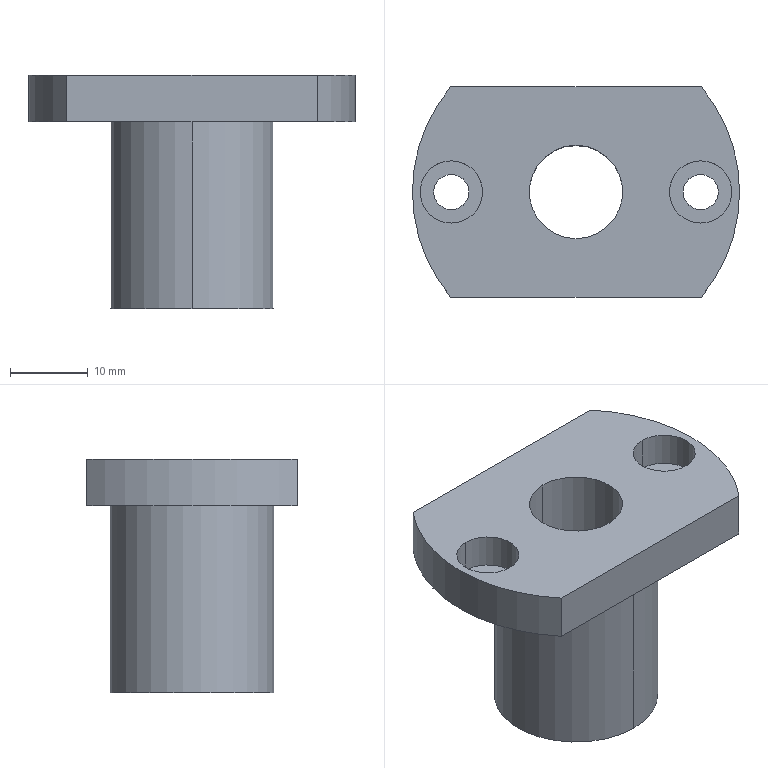Component | SolidWorks | DirectPressureVerticalSeal-1_LMH12UULinearBearing-1 | 1 solid | 21 faces | box 42 x 27 x 30 mm | volume 10727 mm3 | cylinder 14 | plane 7 | commonest cylinder face diameters 8 x4 4.5 x4 12 x2 21 x2 42 x2
build123d program:
from build123d import *

# Parameters (mm, degrees)
BOSS_EXTRUDE1_DEPTH                                 = 6
SKETCH2_W                                           = 24
SKETCH2_H                                           = 10.5
F_12_0_12_DIAMETER_HOLE1_D                          = 12
CYLINDRICAL_COUNTERSUNK_HOLE_FOR_M4_HEX_D           = 4.5
CYLINDRICAL_COUNTERSUNK_HOLE_FOR_M4_HEX_DEPTH       = 30
CYLINDRICAL_COUNTERSUNK_HOLE_FOR_M4_HEX_CBORE_D     = 8
CYLINDRICAL_COUNTERSUNK_HOLE_FOR_M4_HEX_CBORE_DEPTH = 4.4


with BuildPart() as part:
    # Sketch1 → Boss-Extrude1 (new body)
    with BuildSketch(Plane(origin=(6, 0, 0), x_dir=(0, 0, -1), z_dir=(1, 0, 0))):
        with BuildLine():
            Line((13.5, -16.086), (13.5, 16.086))
            ThreePointArc((13.5, 16.086), (0, 21), (-13.5, 16.086))
            Line((-13.5, 16.086), (-13.5, -16.086))
            ThreePointArc((-13.5, -16.086), (0, -21), (13.5, -16.086))
        make_face()
    extrude(amount=-BOSS_EXTRUDE1_DEPTH)

    # Sketch2 → Revolve1 (revolve)
    with BuildSketch(Plane(origin=(0, 0, 0), x_dir=(-1, 0, 0), z_dir=(0, 0, -1)), mode=Mode.PRIVATE) as revolve1_sk:
        with Locations((-18, 5.25)):
            Rectangle(SKETCH2_W, SKETCH2_H)
    revolve(revolve1_sk.sketch.rotate(Axis((30, 0, 0), (-1, 0, 0)), 270), axis=Axis((30, 0, 0), (-1, 0, 0)))

    # 12.0 _12_ Diameter Hole1 (through all)
    with Locations(Plane.ZY):
        with Locations((0, 0)):
            Hole(F_12_0_12_DIAMETER_HOLE1_D / 2)

    # Cylindrical Countersunk Hole for M4 Hex
    with Locations(Plane.ZY):
        with Locations((0, 16), (0, -16)):
            CounterBoreHole(CYLINDRICAL_COUNTERSUNK_HOLE_FOR_M4_HEX_D / 2, CYLINDRICAL_COUNTERSUNK_HOLE_FOR_M4_HEX_CBORE_D / 2, CYLINDRICAL_COUNTERSUNK_HOLE_FOR_M4_HEX_CBORE_DEPTH, depth=CYLINDRICAL_COUNTERSUNK_HOLE_FOR_M4_HEX_DEPTH)


solid = part.part

# Placed as in the assembly
solid = solid.moved(Location((-298.746, 181.873, 324.5), (90, 0, -90)))
STEP:
#1=CARTESIAN_POINT('',(-11.132,7.318,12.602));
#2=VERTEX_POINT('',#1);
#3=CARTESIAN_POINT('',(-11.132,7.003,12.602));
#4=VERTEX_POINT('',#3);
#5=CARTESIAN_POINT('',(-11.132,7.16,12.602));
#6=DIRECTION('',(-0.,-0.,1.));
#7=DIRECTION('',(0.,-1.,0.));
#8=AXIS2_PLACEMENT_3D('',#5,#6,#7);
#9=CIRCLE('',#8,0.1575);
#10=EDGE_CURVE('',#2,#4,#9,.T.);
#11=ORIENTED_EDGE('',*,*,#10,.F.);
#12=CARTESIAN_POINT('',(-11.132,7.318,12.776));
#13=VERTEX_POINT('',#12);
#14=CARTESIAN_POINT('',(-11.132,7.318,12.776));
#15=DIRECTION('',(-0.,-0.,1.));
#16=VECTOR('',#15,39.37);
#17=LINE('',#14,#16);
#18=EDGE_CURVE('',#2,#13,#17,.T.);
#19=ORIENTED_EDGE('',*,*,#18,.T.);
#20=CARTESIAN_POINT('',(-11.132,7.003,12.776));
#21=VERTEX_POINT('',#20);
#22=CARTESIAN_POINT('',(-11.132,7.16,12.776));
#23=DIRECTION('',(-0.,-0.,1.));
#24=DIRECTION('',(0.,-1.,0.));
#25=AXIS2_PLACEMENT_3D('',#22,#23,#24);
#26=CIRCLE('',#25,0.1575);
#27=EDGE_CURVE('',#13,#21,#26,.T.);
#28=ORIENTED_EDGE('',*,*,#27,.T.);
#29=CARTESIAN_POINT('',(-11.132,7.003,12.776));
#30=DIRECTION('',(-0.,-0.,1.));
#31=VECTOR('',#30,39.37);
#32=LINE('',#29,#31);
#33=EDGE_CURVE('',#4,#21,#32,.T.);
#34=ORIENTED_EDGE('',*,*,#33,.F.);
#35=EDGE_LOOP('',(#11,#19,#28,#34));
#36=FACE_OUTER_BOUND('',#35,.T.);
#37=CARTESIAN_POINT('',(-11.132,7.16,12.776));
#38=DIRECTION('',(-0.,-0.,1.));
#39=DIRECTION('',(0.,-1.,0.));
#40=AXIS2_PLACEMENT_3D('',#37,#38,#39);
#41=CYLINDRICAL_SURFACE('',#40,0.1575);
#42=ADVANCED_FACE('',(#36),#41,.F.);
#43=CARTESIAN_POINT('',(-11.132,7.072,12.539));
#44=VERTEX_POINT('',#43);
#45=CARTESIAN_POINT('',(-11.132,7.249,12.539));
#46=VERTEX_POINT('',#45);
#47=CARTESIAN_POINT('',(-11.132,7.16,12.539));
#48=DIRECTION('',(0.,0.,-1.));
#49=DIRECTION('',(0.,1.,0.));
#50=AXIS2_PLACEMENT_3D('',#47,#48,#49);
#51=CIRCLE('',#50,0.08858);
#52=EDGE_CURVE('',#44,#46,#51,.T.);
#53=ORIENTED_EDGE('',*,*,#52,.T.);
#54=CARTESIAN_POINT('',(-11.132,7.249,12.602));
#55=VERTEX_POINT('',#54);
#56=CARTESIAN_POINT('',(-11.132,7.249,12.776));
#57=DIRECTION('',(-0.,-0.,1.));
#58=VECTOR('',#57,39.37);
#59=LINE('',#56,#58);
#60=EDGE_CURVE('',#46,#55,#59,.T.);
#61=ORIENTED_EDGE('',*,*,#60,.T.);
#62=CARTESIAN_POINT('',(-11.132,7.072,12.602));
#63=VERTEX_POINT('',#62);
#64=CARTESIAN_POINT('',(-11.132,7.16,12.602));
#65=DIRECTION('',(-0.,-0.,1.));
#66=DIRECTION('',(0.,-1.,0.));
#67=AXIS2_PLACEMENT_3D('',#64,#65,#66);
#68=CIRCLE('',#67,0.08858);
#69=EDGE_CURVE('',#55,#63,#68,.T.);
#70=ORIENTED_EDGE('',*,*,#69,.T.);
#71=CARTESIAN_POINT('',(-11.132,7.072,12.776));
#72=DIRECTION('',(-0.,-0.,1.));
#73=VECTOR('',#72,39.37);
#74=LINE('',#71,#73);
#75=EDGE_CURVE('',#44,#63,#74,.T.);
#76=ORIENTED_EDGE('',*,*,#75,.F.);
#77=EDGE_LOOP('',(#53,#61,#70,#76));
#78=FACE_OUTER_BOUND('',#77,.T.);
#79=CARTESIAN_POINT('',(-11.132,7.16,12.776));
#80=DIRECTION('',(-0.,-0.,1.));
#81=DIRECTION('',(0.,-1.,0.));
#82=AXIS2_PLACEMENT_3D('',#79,#80,#81);
#83=CYLINDRICAL_SURFACE('',#82,0.08858);
#84=ADVANCED_FACE('',(#78),#83,.F.);
#85=CARTESIAN_POINT('',(-12.392,7.318,12.602));
#86=VERTEX_POINT('',#85);
#87=CARTESIAN_POINT('',(-12.392,7.003,12.602));
#88=VERTEX_POINT('',#87);
#89=CARTESIAN_POINT('',(-12.392,7.16,12.602));
#90=DIRECTION('',(-0.,-0.,1.));
#91=DIRECTION('',(0.,-1.,0.));
#92=AXIS2_PLACEMENT_3D('',#89,#90,#91);
#93=CIRCLE('',#92,0.1575);
#94=EDGE_CURVE('',#86,#88,#93,.T.);
#95=ORIENTED_EDGE('',*,*,#94,.F.);
#96=CARTESIAN_POINT('',(-12.392,7.318,12.776));
#97=VERTEX_POINT('',#96);
#98=CARTESIAN_POINT('',(-12.392,7.318,12.776));
#99=DIRECTION('',(-0.,-0.,1.));
#100=VECTOR('',#99,39.37);
#101=LINE('',#98,#100);
#102=EDGE_CURVE('',#86,#97,#101,.T.);
#103=ORIENTED_EDGE('',*,*,#102,.T.);
#104=CARTESIAN_POINT('',(-12.392,7.003,12.776));
#105=VERTEX_POINT('',#104);
#106=CARTESIAN_POINT('',(-12.392,7.16,12.776));
#107=DIRECTION('',(-0.,-0.,1.));
#108=DIRECTION('',(0.,-1.,0.));
#109=AXIS2_PLACEMENT_3D('',#106,#107,#108);
#110=CIRCLE('',#109,0.1575);
#111=EDGE_CURVE('',#97,#105,#110,.T.);
#112=ORIENTED_EDGE('',*,*,#111,.T.);
#113=CARTESIAN_POINT('',(-12.392,7.003,12.776));
#114=DIRECTION('',(-0.,-0.,1.));
#115=VECTOR('',#114,39.37);
#116=LINE('',#113,#115);
#117=EDGE_CURVE('',#88,#105,#116,.T.);
#118=ORIENTED_EDGE('',*,*,#117,.F.);
#119=EDGE_LOOP('',(#95,#103,#112,#118));
#120=FACE_OUTER_BOUND('',#119,.T.);
#121=CARTESIAN_POINT('',(-12.392,7.16,12.776));
#122=DIRECTION('',(-0.,-0.,1.));
#123=DIRECTION('',(0.,-1.,0.));
#124=AXIS2_PLACEMENT_3D('',#121,#122,#123);
#125=CYLINDRICAL_SURFACE('',#124,0.1575);
#126=ADVANCED_FACE('',(#120),#125,.F.);
#127=CARTESIAN_POINT('',(-12.392,7.072,12.539));
#128=VERTEX_POINT('',#127);
#129=CARTESIAN_POINT('',(-12.392,7.249,12.539));
#130=VERTEX_POINT('',#129);
#131=CARTESIAN_POINT('',(-12.392,7.16,12.539));
#132=DIRECTION('',(0.,0.,-1.));
#133=DIRECTION('',(0.,1.,0.));
#134=AXIS2_PLACEMENT_3D('',#131,#132,#133);
#135=CIRCLE('',#134,0.08858);
#136=EDGE_CURVE('',#128,#130,#135,.T.);
#137=ORIENTED_EDGE('',*,*,#136,.T.);
#138=CARTESIAN_POINT('',(-12.392,7.249,12.602));
#139=VERTEX_POINT('',#138);
#140=CARTESIAN_POINT('',(-12.392,7.249,12.776));
#141=DIRECTION('',(-0.,-0.,1.));
#142=VECTOR('',#141,39.37);
#143=LINE('',#140,#142);
#144=EDGE_CURVE('',#130,#139,#143,.T.);
#145=ORIENTED_EDGE('',*,*,#144,.T.);
#146=CARTESIAN_POINT('',(-12.392,7.072,12.602));
#147=VERTEX_POINT('',#146);
#148=CARTESIAN_POINT('',(-12.392,7.16,12.602));
#149=DIRECTION('',(-0.,-0.,1.));
#150=DIRECTION('',(0.,-1.,0.));
#151=AXIS2_PLACEMENT_3D('',#148,#149,#150);
#152=CIRCLE('',#151,0.08858);
#153=EDGE_CURVE('',#139,#147,#152,.T.);
#154=ORIENTED_EDGE('',*,*,#153,.T.);
#155=CARTESIAN_POINT('',(-12.392,7.072,12.776));
#156=DIRECTION('',(-0.,-0.,1.));
#157=VECTOR('',#156,39.37);
#158=LINE('',#155,#157);
#159=EDGE_CURVE('',#128,#147,#158,.T.);
#160=ORIENTED_EDGE('',*,*,#159,.F.);
#161=EDGE_LOOP('',(#137,#145,#154,#160));
#162=FACE_OUTER_BOUND('',#161,.T.);
#163=CARTESIAN_POINT('',(-12.392,7.16,12.776));
#164=DIRECTION('',(-0.,-0.,1.));
#165=DIRECTION('',(0.,-1.,0.));
#166=AXIS2_PLACEMENT_3D('',#163,#164,#165);
#167=CYLINDRICAL_SURFACE('',#166,0.08858);
#168=ADVANCED_FACE('',(#162),#167,.F.);
#169=CARTESIAN_POINT('',(-11.762,7.397,11.594));
#170=VERTEX_POINT('',#169);
#171=CARTESIAN_POINT('',(-11.762,6.924,11.594));
#172=VERTEX_POINT('',#171);
#173=CARTESIAN_POINT('',(-11.762,7.16,11.594));
#174=DIRECTION('',(-0.,-0.,1.));
#175=DIRECTION('',(0.,-1.,0.));
#176=AXIS2_PLACEMENT_3D('',#173,#174,#175);
#177=CIRCLE('',#176,0.2362);
#178=EDGE_CURVE('',#170,#172,#177,.T.);
#179=ORIENTED_EDGE('',*,*,#178,.F.);
#180=CARTESIAN_POINT('',(-11.762,7.397,12.776));
#181=VERTEX_POINT('',#180);
#182=CARTESIAN_POINT('',(-11.762,7.397,12.776));
#183=DIRECTION('',(-0.,-0.,1.));
#184=VECTOR('',#183,39.37);
#185=LINE('',#182,#184);
#186=EDGE_CURVE('',#170,#181,#185,.T.);
#187=ORIENTED_EDGE('',*,*,#186,.T.);
#188=CARTESIAN_POINT('',(-11.762,6.924,12.776));
#189=VERTEX_POINT('',#188);
#190=CARTESIAN_POINT('',(-11.762,7.16,12.776));
#191=DIRECTION('',(-0.,-0.,1.));
#192=DIRECTION('',(0.,-1.,0.));
#193=AXIS2_PLACEMENT_3D('',#190,#191,#192);
#194=CIRCLE('',#193,0.2362);
#195=EDGE_CURVE('',#181,#189,#194,.T.);
#196=ORIENTED_EDGE('',*,*,#195,.T.);
#197=CARTESIAN_POINT('',(-11.762,6.924,12.776));
#198=DIRECTION('',(-0.,-0.,1.));
#199=VECTOR('',#198,39.37);
#200=LINE('',#197,#199);
#201=EDGE_CURVE('',#172,#189,#200,.T.);
#202=ORIENTED_EDGE('',*,*,#201,.F.);
#203=EDGE_LOOP('',(#179,#187,#196,#202));
#204=FACE_OUTER_BOUND('',#203,.T.);
#205=CARTESIAN_POINT('',(-11.762,7.16,12.776));
#206=DIRECTION('',(-0.,-0.,1.));
#207=DIRECTION('',(0.,-1.,0.));
#208=AXIS2_PLACEMENT_3D('',#205,#206,#207);
#209=CYLINDRICAL_SURFACE('',#208,0.2362);
#210=ADVANCED_FACE('',(#204),#209,.F.);
#211=CARTESIAN_POINT('',(-11.762,6.747,11.594));
#212=VERTEX_POINT('',#211);
#213=CARTESIAN_POINT('',(-11.762,7.574,11.594));
#214=VERTEX_POINT('',#213);
#215=CARTESIAN_POINT('',(-11.762,7.16,11.594));
#216=DIRECTION('',(-0.,-0.,1.));
#217=DIRECTION('',(0.,-1.,0.));
#218=AXIS2_PLACEMENT_3D('',#215,#216,#217);
#219=CIRCLE('',#218,0.4134);
#220=EDGE_CURVE('',#212,#214,#219,.T.);
#221=ORIENTED_EDGE('',*,*,#220,.T.);
#222=CARTESIAN_POINT('',(-11.762,7.574,12.539));
#223=VERTEX_POINT('',#222);
#224=CARTESIAN_POINT('',(-11.762,7.574,11.594));
#225=DIRECTION('',(-0.,-0.,1.));
#226=VECTOR('',#225,39.37);
#227=LINE('',#224,#226);
#228=EDGE_CURVE('',#214,#223,#227,.T.);
#229=ORIENTED_EDGE('',*,*,#228,.T.);
#230=CARTESIAN_POINT('',(-11.762,6.747,12.539));
#231=VERTEX_POINT('',#230);
#232=CARTESIAN_POINT('',(-11.762,7.16,12.539));
#233=DIRECTION('',(-0.,-0.,1.));
#234=DIRECTION('',(0.,-1.,0.));
#235=AXIS2_PLACEMENT_3D('',#232,#233,#234);
#236=CIRCLE('',#235,0.4134);
#237=EDGE_CURVE('',#231,#223,#236,.T.);
#238=ORIENTED_EDGE('',*,*,#237,.F.);
#239=CARTESIAN_POINT('',(-11.762,6.747,11.594));
#240=DIRECTION('',(-0.,-0.,1.));
#241=VECTOR('',#240,39.37);
#242=LINE('',#239,#241);
#243=EDGE_CURVE('',#212,#231,#242,.T.);
#244=ORIENTED_EDGE('',*,*,#243,.F.);
#245=EDGE_LOOP('',(#221,#229,#238,#244));
#246=FACE_OUTER_BOUND('',#245,.T.);
#247=CARTESIAN_POINT('',(-11.762,7.16,11.594));
#248=DIRECTION('',(-0.,-0.,1.));
#249=DIRECTION('',(0.,-1.,0.));
#250=AXIS2_PLACEMENT_3D('',#247,#248,#249);
#251=CYLINDRICAL_SURFACE('',#250,0.4134);
#252=ADVANCED_FACE('',(#246),#251,.T.);
#253=CARTESIAN_POINT('',(-12.395,6.629,12.539));
#254=VERTEX_POINT('',#253);
#255=CARTESIAN_POINT('',(-12.395,7.692,12.539));
#256=VERTEX_POINT('',#255);
#257=CARTESIAN_POINT('',(-11.762,7.16,12.539));
#258=DIRECTION('',(0.,0.,-1.));
#259=DIRECTION('',(0.,1.,0.));
#260=AXIS2_PLACEMENT_3D('',#257,#258,#259);
#261=CIRCLE('',#260,0.8268);
#262=EDGE_CURVE('',#254,#256,#261,.T.);
#263=ORIENTED_EDGE('',*,*,#262,.F.);
#264=CARTESIAN_POINT('',(-12.395,6.629,12.776));
#265=VERTEX_POINT('',#264);
#266=CARTESIAN_POINT('',(-12.395,6.629,12.776));
#267=DIRECTION('',(0.,0.,-1.));
#268=VECTOR('',#267,39.37);
#269=LINE('',#266,#268);
#270=EDGE_CURVE('',#265,#254,#269,.T.);
#271=ORIENTED_EDGE('',*,*,#270,.F.);
#272=CARTESIAN_POINT('',(-12.395,7.692,12.776));
#273=VERTEX_POINT('',#272);
#274=CARTESIAN_POINT('',(-11.762,7.16,12.776));
#275=DIRECTION('',(0.,0.,-1.));
#276=DIRECTION('',(0.,1.,0.));
#277=AXIS2_PLACEMENT_3D('',#274,#275,#276);
#278=CIRCLE('',#277,0.8268);
#279=EDGE_CURVE('',#265,#273,#278,.T.);
#280=ORIENTED_EDGE('',*,*,#279,.T.);
#281=CARTESIAN_POINT('',(-12.395,7.692,12.776));
#282=DIRECTION('',(0.,0.,-1.));
#283=VECTOR('',#282,39.37);
#284=LINE('',#281,#283);
#285=EDGE_CURVE('',#273,#256,#284,.T.);
#286=ORIENTED_EDGE('',*,*,#285,.T.);
#287=EDGE_LOOP('',(#263,#271,#280,#286));
#288=FACE_OUTER_BOUND('',#287,.T.);
#289=CARTESIAN_POINT('',(-11.762,7.16,12.776));
#290=DIRECTION('',(0.,0.,-1.));
#291=DIRECTION('',(0.,1.,0.));
#292=AXIS2_PLACEMENT_3D('',#289,#290,#291);
#293=CYLINDRICAL_SURFACE('',#292,0.8268);
#294=ADVANCED_FACE('',(#288),#293,.T.);
#295=CARTESIAN_POINT('',(-11.128,6.629,12.539));
#296=VERTEX_POINT('',#295);
#297=CARTESIAN_POINT('',(-11.128,6.629,12.539));
#298=DIRECTION('',(-1.,-0.,-0.));
#299=VECTOR('',#298,39.37);
#300=LINE('',#297,#299);
#301=EDGE_CURVE('',#296,#254,#300,.T.);
#302=ORIENTED_EDGE('',*,*,#301,.F.);
#303=CARTESIAN_POINT('',(-11.128,6.629,12.776));
#304=VERTEX_POINT('',#303);
#305=CARTESIAN_POINT('',(-11.128,6.629,12.776));
#306=DIRECTION('',(0.,0.,-1.));
#307=VECTOR('',#306,39.37);
#308=LINE('',#305,#307);
#309=EDGE_CURVE('',#304,#296,#308,.T.);
#310=ORIENTED_EDGE('',*,*,#309,.F.);
#311=CARTESIAN_POINT('',(-11.128,6.629,12.776));
#312=DIRECTION('',(-1.,-0.,-0.));
#313=VECTOR('',#312,39.37);
#314=LINE('',#311,#313);
#315=EDGE_CURVE('',#304,#265,#314,.T.);
#316=ORIENTED_EDGE('',*,*,#315,.T.);
#317=ORIENTED_EDGE('',*,*,#270,.T.);
#318=EDGE_LOOP('',(#302,#310,#316,#317));
#319=FACE_OUTER_BOUND('',#318,.T.);
#320=CARTESIAN_POINT('',(-11.128,6.629,12.776));
#321=DIRECTION('',(0.,-1.,-0.));
#322=DIRECTION('',(0.,0.,-1.));
#323=AXIS2_PLACEMENT_3D('',#320,#321,#322);
#324=PLANE('',#323);
#325=ADVANCED_FACE('',(#319),#324,.T.);
#326=CARTESIAN_POINT('',(-11.128,7.692,12.539));
#327=VERTEX_POINT('',#326);
#328=CARTESIAN_POINT('',(-11.762,7.16,12.539));
#329=DIRECTION('',(0.,0.,-1.));
#330=DIRECTION('',(0.,1.,0.));
#331=AXIS2_PLACEMENT_3D('',#328,#329,#330);
#332=CIRCLE('',#331,0.8268);
#333=EDGE_CURVE('',#327,#296,#332,.T.);
#334=ORIENTED_EDGE('',*,*,#333,.F.);
#335=CARTESIAN_POINT('',(-11.128,7.692,12.776));
#336=VERTEX_POINT('',#335);
#337=CARTESIAN_POINT('',(-11.128,7.692,12.776));
#338=DIRECTION('',(0.,0.,-1.));
#339=VECTOR('',#338,39.37);
#340=LINE('',#337,#339);
#341=EDGE_CURVE('',#336,#327,#340,.T.);
#342=ORIENTED_EDGE('',*,*,#341,.F.);
#343=CARTESIAN_POINT('',(-11.762,7.16,12.776));
#344=DIRECTION('',(0.,0.,-1.));
#345=DIRECTION('',(0.,1.,0.));
#346=AXIS2_PLACEMENT_3D('',#343,#344,#345);
#347=CIRCLE('',#346,0.8268);
#348=EDGE_CURVE('',#336,#304,#347,.T.);
#349=ORIENTED_EDGE('',*,*,#348,.T.);
#350=ORIENTED_EDGE('',*,*,#309,.T.);
#351=EDGE_LOOP('',(#334,#342,#349,#350));
#352=FACE_OUTER_BOUND('',#351,.T.);
#353=CARTESIAN_POINT('',(-11.762,7.16,12.776));
#354=DIRECTION('',(0.,0.,-1.));
#355=DIRECTION('',(0.,1.,0.));
#356=AXIS2_PLACEMENT_3D('',#353,#354,#355);
#357=CYLINDRICAL_SURFACE('',#356,0.8268);
#358=ADVANCED_FACE('',(#352),#357,.T.);
#359=CARTESIAN_POINT('',(-12.395,7.692,12.539));
#360=DIRECTION('',(1.,0.,0.));
#361=VECTOR('',#360,39.37);
#362=LINE('',#359,#361);
#363=EDGE_CURVE('',#256,#327,#362,.T.);
#364=ORIENTED_EDGE('',*,*,#363,.F.);
#365=ORIENTED_EDGE('',*,*,#285,.F.);
#366=CARTESIAN_POINT('',(-12.395,7.692,12.776));
#367=DIRECTION('',(1.,0.,0.));
#368=VECTOR('',#367,39.37);
#369=LINE('',#366,#368);
#370=EDGE_CURVE('',#273,#336,#369,.T.);
#371=ORIENTED_EDGE('',*,*,#370,.T.);
#372=ORIENTED_EDGE('',*,*,#341,.T.);
#373=EDGE_LOOP('',(#364,#365,#371,#372));
#374=FACE_OUTER_BOUND('',#373,.T.);
#375=CARTESIAN_POINT('',(-12.395,7.692,12.776));
#376=DIRECTION('',(-0.,1.,0.));
#377=DIRECTION('',(1.,0.,0.));
#378=AXIS2_PLACEMENT_3D('',#375,#376,#377);
#379=PLANE('',#378);
#380=ADVANCED_FACE('',(#374),#379,.T.);
#381=CARTESIAN_POINT('',(-11.132,7.16,12.776));
#382=DIRECTION('',(-0.,-0.,1.));
#383=DIRECTION('',(0.,-1.,0.));
#384=AXIS2_PLACEMENT_3D('',#381,#382,#383);
#385=CIRCLE('',#384,0.1575);
#386=EDGE_CURVE('',#21,#13,#385,.T.);
#387=ORIENTED_EDGE('',*,*,#386,.F.);
#388=ORIENTED_EDGE('',*,*,#27,.F.);
#389=EDGE_LOOP('',(#387,#388));
#390=FACE_BOUND('',#389,.T.);
#391=CARTESIAN_POINT('',(-12.392,7.16,12.776));
#392=DIRECTION('',(-0.,-0.,1.));
#393=DIRECTION('',(0.,-1.,0.));
#394=AXIS2_PLACEMENT_3D('',#391,#392,#393);
#395=CIRCLE('',#394,0.1575);
#396=EDGE_CURVE('',#105,#97,#395,.T.);
#397=ORIENTED_EDGE('',*,*,#396,.F.);
#398=ORIENTED_EDGE('',*,*,#111,.F.);
#399=EDGE_LOOP('',(#397,#398));
#400=FACE_BOUND('',#399,.T.);
#401=CARTESIAN_POINT('',(-11.762,7.16,12.776));
#402=DIRECTION('',(-0.,-0.,1.));
#403=DIRECTION('',(0.,-1.,0.));
#404=AXIS2_PLACEMENT_3D('',#401,#402,#403);
#405=CIRCLE('',#404,0.2362);
#406=EDGE_CURVE('',#189,#181,#405,.T.);
#407=ORIENTED_EDGE('',*,*,#406,.F.);
#408=ORIENTED_EDGE('',*,*,#195,.F.);
#409=EDGE_LOOP('',(#407,#408));
#410=FACE_BOUND('',#409,.T.);
#411=ORIENTED_EDGE('',*,*,#279,.F.);
#412=ORIENTED_EDGE('',*,*,#315,.F.);
#413=ORIENTED_EDGE('',*,*,#348,.F.);
#414=ORIENTED_EDGE('',*,*,#370,.F.);
#415=EDGE_LOOP('',(#411,#412,#413,#414));
#416=FACE_OUTER_BOUND('',#415,.T.);
#417=CARTESIAN_POINT('',(-11.762,7.16,12.776));
#418=DIRECTION('',(0.,0.,-1.));
#419=DIRECTION('',(-0.,1.,0.));
#420=AXIS2_PLACEMENT_3D('',#417,#418,#419);
#421=PLANE('',#420);
#422=ADVANCED_FACE('',(#390,#400,#410,#416),#421,.F.);
#423=ORIENTED_EDGE('',*,*,#52,.F.);
#424=CARTESIAN_POINT('',(-11.132,7.16,12.539));
#425=DIRECTION('',(0.,0.,-1.));
#426=DIRECTION('',(0.,1.,0.));
#427=AXIS2_PLACEMENT_3D('',#424,#425,#426);
#428=CIRCLE('',#427,0.08858);
#429=EDGE_CURVE('',#46,#44,#428,.T.);
#430=ORIENTED_EDGE('',*,*,#429,.F.);
#431=EDGE_LOOP('',(#423,#430));
#432=FACE_BOUND('',#431,.T.);
#433=ORIENTED_EDGE('',*,*,#136,.F.);
#434=CARTESIAN_POINT('',(-12.392,7.16,12.539));
#435=DIRECTION('',(0.,0.,-1.));
#436=DIRECTION('',(0.,1.,0.));
#437=AXIS2_PLACEMENT_3D('',#434,#435,#436);
#438=CIRCLE('',#437,0.08858);
#439=EDGE_CURVE('',#130,#128,#438,.T.);
#440=ORIENTED_EDGE('',*,*,#439,.F.);
#441=EDGE_LOOP('',(#433,#440));
#442=FACE_BOUND('',#441,.T.);
#443=ORIENTED_EDGE('',*,*,#237,.T.);
#444=CARTESIAN_POINT('',(-11.762,7.16,12.539));
#445=DIRECTION('',(-0.,-0.,1.));
#446=DIRECTION('',(0.,-1.,0.));
#447=AXIS2_PLACEMENT_3D('',#444,#445,#446);
#448=CIRCLE('',#447,0.4134);
#449=EDGE_CURVE('',#223,#231,#448,.T.);
#450=ORIENTED_EDGE('',*,*,#449,.T.);
#451=EDGE_LOOP('',(#443,#450));
#452=FACE_BOUND('',#451,.T.);
#453=ORIENTED_EDGE('',*,*,#262,.T.);
#454=ORIENTED_EDGE('',*,*,#363,.T.);
#455=ORIENTED_EDGE('',*,*,#333,.T.);
#456=ORIENTED_EDGE('',*,*,#301,.T.);
#457=EDGE_LOOP('',(#453,#454,#455,#456));
#458=FACE_OUTER_BOUND('',#457,.T.);
#459=CARTESIAN_POINT('',(-11.762,7.16,12.539));
#460=DIRECTION('',(0.,0.,-1.));
#461=DIRECTION('',(-0.,1.,0.));
#462=AXIS2_PLACEMENT_3D('',#459,#460,#461);
#463=PLANE('',#462);
#464=ADVANCED_FACE('',(#432,#442,#452,#458),#463,.T.);
#465=ORIENTED_EDGE('',*,*,#228,.F.);
#466=CARTESIAN_POINT('',(-11.762,7.16,11.594));
#467=DIRECTION('',(-0.,-0.,1.));
#468=DIRECTION('',(0.,-1.,0.));
#469=AXIS2_PLACEMENT_3D('',#466,#467,#468);
#470=CIRCLE('',#469,0.4134);
#471=EDGE_CURVE('',#214,#212,#470,.T.);
#472=ORIENTED_EDGE('',*,*,#471,.T.);
#473=ORIENTED_EDGE('',*,*,#243,.T.);
#474=ORIENTED_EDGE('',*,*,#449,.F.);
#475=EDGE_LOOP('',(#465,#472,#473,#474));
#476=FACE_OUTER_BOUND('',#475,.T.);
#477=CARTESIAN_POINT('',(-11.762,7.16,11.594));
#478=DIRECTION('',(-0.,-0.,1.));
#479=DIRECTION('',(0.,-1.,0.));
#480=AXIS2_PLACEMENT_3D('',#477,#478,#479);
#481=CYLINDRICAL_SURFACE('',#480,0.4134);
#482=ADVANCED_FACE('',(#476),#481,.T.);
#483=CARTESIAN_POINT('',(-11.762,7.16,11.594));
#484=DIRECTION('',(-0.,-0.,1.));
#485=DIRECTION('',(0.,-1.,0.));
#486=AXIS2_PLACEMENT_3D('',#483,#484,#485);
#487=CIRCLE('',#486,0.2362);
#488=EDGE_CURVE('',#172,#170,#487,.T.);
#489=ORIENTED_EDGE('',*,*,#488,.T.);
#490=ORIENTED_EDGE('',*,*,#178,.T.);
#491=EDGE_LOOP('',(#489,#490));
#492=FACE_BOUND('',#491,.T.);
#493=ORIENTED_EDGE('',*,*,#220,.F.);
#494=ORIENTED_EDGE('',*,*,#471,.F.);
#495=EDGE_LOOP('',(#493,#494));
#496=FACE_OUTER_BOUND('',#495,.T.);
#497=CARTESIAN_POINT('',(-11.348,7.16,11.594));
#498=DIRECTION('',(0.,0.,-1.));
#499=DIRECTION('',(-0.,1.,0.));
#500=AXIS2_PLACEMENT_3D('',#497,#498,#499);
#501=PLANE('',#500);
#502=ADVANCED_FACE('',(#492,#496),#501,.T.);
#503=ORIENTED_EDGE('',*,*,#186,.F.);
#504=ORIENTED_EDGE('',*,*,#488,.F.);
#505=ORIENTED_EDGE('',*,*,#201,.T.);
#506=ORIENTED_EDGE('',*,*,#406,.T.);
#507=EDGE_LOOP('',(#503,#504,#505,#506));
#508=FACE_OUTER_BOUND('',#507,.T.);
#509=CARTESIAN_POINT('',(-11.762,7.16,12.776));
#510=DIRECTION('',(-0.,-0.,1.));
#511=DIRECTION('',(0.,-1.,0.));
#512=AXIS2_PLACEMENT_3D('',#509,#510,#511);
#513=CYLINDRICAL_SURFACE('',#512,0.2362);
#514=ADVANCED_FACE('',(#508),#513,.F.);
#515=ORIENTED_EDGE('',*,*,#144,.F.);
#516=ORIENTED_EDGE('',*,*,#439,.T.);
#517=ORIENTED_EDGE('',*,*,#159,.T.);
#518=CARTESIAN_POINT('',(-12.392,7.16,12.602));
#519=DIRECTION('',(-0.,-0.,1.));
#520=DIRECTION('',(0.,-1.,0.));
#521=AXIS2_PLACEMENT_3D('',#518,#519,#520);
#522=CIRCLE('',#521,0.08858);
#523=EDGE_CURVE('',#147,#139,#522,.T.);
#524=ORIENTED_EDGE('',*,*,#523,.T.);
#525=EDGE_LOOP('',(#515,#516,#517,#524));
#526=FACE_OUTER_BOUND('',#525,.T.);
#527=CARTESIAN_POINT('',(-12.392,7.16,12.776));
#528=DIRECTION('',(-0.,-0.,1.));
#529=DIRECTION('',(0.,-1.,0.));
#530=AXIS2_PLACEMENT_3D('',#527,#528,#529);
#531=CYLINDRICAL_SURFACE('',#530,0.08858);
#532=ADVANCED_FACE('',(#526),#531,.F.);
#533=ORIENTED_EDGE('',*,*,#523,.F.);
#534=ORIENTED_EDGE('',*,*,#153,.F.);
#535=EDGE_LOOP('',(#533,#534));
#536=FACE_BOUND('',#535,.T.);
#537=CARTESIAN_POINT('',(-12.392,7.16,12.602));
#538=DIRECTION('',(-0.,-0.,1.));
#539=DIRECTION('',(0.,-1.,0.));
#540=AXIS2_PLACEMENT_3D('',#537,#538,#539);
#541=CIRCLE('',#540,0.1575);
#542=EDGE_CURVE('',#88,#86,#541,.T.);
#543=ORIENTED_EDGE('',*,*,#542,.T.);
#544=ORIENTED_EDGE('',*,*,#94,.T.);
#545=EDGE_LOOP('',(#543,#544));
#546=FACE_OUTER_BOUND('',#545,.T.);
#547=CARTESIAN_POINT('',(-12.303,7.16,12.602));
#548=DIRECTION('',(0.,0.,-1.));
#549=DIRECTION('',(-0.,1.,0.));
#550=AXIS2_PLACEMENT_3D('',#547,#548,#549);
#551=PLANE('',#550);
#552=ADVANCED_FACE('',(#536,#546),#551,.F.);
#553=ORIENTED_EDGE('',*,*,#102,.F.);
#554=ORIENTED_EDGE('',*,*,#542,.F.);
#555=ORIENTED_EDGE('',*,*,#117,.T.);
#556=ORIENTED_EDGE('',*,*,#396,.T.);
#557=EDGE_LOOP('',(#553,#554,#555,#556));
#558=FACE_OUTER_BOUND('',#557,.T.);
#559=CARTESIAN_POINT('',(-12.392,7.16,12.776));
#560=DIRECTION('',(-0.,-0.,1.));
#561=DIRECTION('',(0.,-1.,0.));
#562=AXIS2_PLACEMENT_3D('',#559,#560,#561);
#563=CYLINDRICAL_SURFACE('',#562,0.1575);
#564=ADVANCED_FACE('',(#558),#563,.F.);
#565=ORIENTED_EDGE('',*,*,#60,.F.);
#566=ORIENTED_EDGE('',*,*,#429,.T.);
#567=ORIENTED_EDGE('',*,*,#75,.T.);
#568=CARTESIAN_POINT('',(-11.132,7.16,12.602));
#569=DIRECTION('',(-0.,-0.,1.));
#570=DIRECTION('',(0.,-1.,0.));
#571=AXIS2_PLACEMENT_3D('',#568,#569,#570);
#572=CIRCLE('',#571,0.08858);
#573=EDGE_CURVE('',#63,#55,#572,.T.);
#574=ORIENTED_EDGE('',*,*,#573,.T.);
#575=EDGE_LOOP('',(#565,#566,#567,#574));
#576=FACE_OUTER_BOUND('',#575,.T.);
#577=CARTESIAN_POINT('',(-11.132,7.16,12.776));
#578=DIRECTION('',(-0.,-0.,1.));
#579=DIRECTION('',(0.,-1.,0.));
#580=AXIS2_PLACEMENT_3D('',#577,#578,#579);
#581=CYLINDRICAL_SURFACE('',#580,0.08858);
#582=ADVANCED_FACE('',(#576),#581,.F.);
#583=ORIENTED_EDGE('',*,*,#573,.F.);
#584=ORIENTED_EDGE('',*,*,#69,.F.);
#585=EDGE_LOOP('',(#583,#584));
#586=FACE_BOUND('',#585,.T.);
#587=CARTESIAN_POINT('',(-11.132,7.16,12.602));
#588=DIRECTION('',(-0.,-0.,1.));
#589=DIRECTION('',(0.,-1.,0.));
#590=AXIS2_PLACEMENT_3D('',#587,#588,#589);
#591=CIRCLE('',#590,0.1575);
#592=EDGE_CURVE('',#4,#2,#591,.T.);
#593=ORIENTED_EDGE('',*,*,#592,.T.);
#594=ORIENTED_EDGE('',*,*,#10,.T.);
#595=EDGE_LOOP('',(#593,#594));
#596=FACE_OUTER_BOUND('',#595,.T.);
#597=CARTESIAN_POINT('',(-11.043,7.16,12.602));
#598=DIRECTION('',(0.,0.,-1.));
#599=DIRECTION('',(-0.,1.,0.));
#600=AXIS2_PLACEMENT_3D('',#597,#598,#599);
#601=PLANE('',#600);
#602=ADVANCED_FACE('',(#586,#596),#601,.F.);
#603=ORIENTED_EDGE('',*,*,#18,.F.);
#604=ORIENTED_EDGE('',*,*,#592,.F.);
#605=ORIENTED_EDGE('',*,*,#33,.T.);
#606=ORIENTED_EDGE('',*,*,#386,.T.);
#607=EDGE_LOOP('',(#603,#604,#605,#606));
#608=FACE_OUTER_BOUND('',#607,.T.);
#609=CARTESIAN_POINT('',(-11.132,7.16,12.776));
#610=DIRECTION('',(-0.,-0.,1.));
#611=DIRECTION('',(0.,-1.,0.));
#612=AXIS2_PLACEMENT_3D('',#609,#610,#611);
#613=CYLINDRICAL_SURFACE('',#612,0.1575);
#614=ADVANCED_FACE('',(#608),#613,.F.);
#615=CLOSED_SHELL('',(#42,#84,#126,#168,#210,#252,#294,#325,#358,#380,#422,#464,#482,#502,#514,#532,#552,#564,#582,#602,#614));
#616=MANIFOLD_SOLID_BREP('',#615);
#617=CARTESIAN_POINT('',(0.,0.,0.));
#618=DIRECTION('',(0.,0.,1.));
#619=DIRECTION('',(1.,0.,0.));
#620=AXIS2_PLACEMENT_3D('',#617,#618,#619);
#621=(LENGTH_UNIT()NAMED_UNIT(*)SI_UNIT($,.METRE.));
#622=LENGTH_MEASURE_WITH_UNIT(LENGTH_MEASURE(0.0254),#621);
#623=DIMENSIONAL_EXPONENTS(1.,0.,0.,0.,0.,0.,0.);
#624=(CONVERSION_BASED_UNIT('',#622)LENGTH_UNIT()NAMED_UNIT(#623));
#625=UNCERTAINTY_MEASURE_WITH_UNIT(LENGTH_MEASURE(0.00001),#624,'','');
#626=(NAMED_UNIT(*)PLANE_ANGLE_UNIT()SI_UNIT($,.RADIAN.));
#627=(NAMED_UNIT(*)SI_UNIT($,.STERADIAN.)SOLID_ANGLE_UNIT());
#628=(GEOMETRIC_REPRESENTATION_CONTEXT(3)GLOBAL_UNCERTAINTY_ASSIGNED_CONTEXT((#625))GLOBAL_UNIT_ASSIGNED_CONTEXT((#624,#626,#627))REPRESENTATION_CONTEXT('',''));
#629=ADVANCED_BREP_SHAPE_REPRESENTATION('',(#616,#620),#628);
#630=COLOUR_RGB('',0.7922,0.8196,0.9333);
#631=FILL_AREA_STYLE_COLOUR('',#630);
#632=FILL_AREA_STYLE('',(#631));
#633=SURFACE_STYLE_FILL_AREA(#632);
#634=SURFACE_SIDE_STYLE('',(#633));
#635=SURFACE_STYLE_USAGE(.BOTH.,#634);
#636=PRESENTATION_STYLE_ASSIGNMENT((#635));
#637=STYLED_ITEM('',(#636),#616);
#638=PRESENTATION_LAYER_ASSIGNMENT('','',(#637));
#639=(LENGTH_UNIT()NAMED_UNIT(*)SI_UNIT($,.METRE.));
#640=LENGTH_MEASURE_WITH_UNIT(LENGTH_MEASURE(0.0254),#639);
#641=DIMENSIONAL_EXPONENTS(1.,0.,0.,0.,0.,0.,0.);
#642=(CONVERSION_BASED_UNIT('',#640)LENGTH_UNIT()NAMED_UNIT(#641));
#643=UNCERTAINTY_MEASURE_WITH_UNIT(LENGTH_MEASURE(0.00001),#642,'','');
#644=(NAMED_UNIT(*)PLANE_ANGLE_UNIT()SI_UNIT($,.RADIAN.));
#645=(NAMED_UNIT(*)SI_UNIT($,.STERADIAN.)SOLID_ANGLE_UNIT());
#646=(GEOMETRIC_REPRESENTATION_CONTEXT(3)GLOBAL_UNCERTAINTY_ASSIGNED_CONTEXT((#643))GLOBAL_UNIT_ASSIGNED_CONTEXT((#642,#644,#645))REPRESENTATION_CONTEXT('',''));
#647=MECHANICAL_DESIGN_GEOMETRIC_PRESENTATION_REPRESENTATION('',(#637),#646);